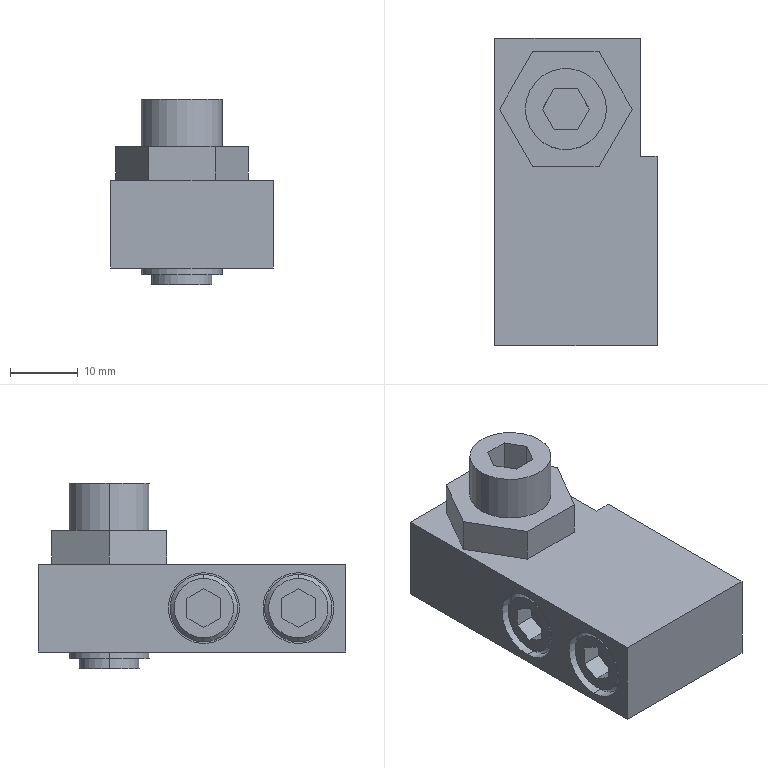Component | SolidWorks | SMC-MXS20-100AS-M9N-1_0SMC-MXS20-100AS-M9N-4-1 | 1 solid | 61 faces | box 24 x 45.5 x 27.5 mm | volume 15366 mm3 | plane 43 | cylinder 14 | cone 4 | commonest cylinder face diameters 10 x4 10.5 x4 12 x4 8.9 x2
build123d program:
from build123d import *

# Parameters (mm, degrees)
BOSS_EXTRUDE1_DEPTH      = 6.5
BOSS_EXTRUDE1_DEPTH_BACK = 6.5
SKETCH2_W                = 13
SKETCH2_H                = 6
CUT_EXTRUDE1_DEPTH       = 6
SKETCH5_R                = 6
BOSS_EXTRUDE2_DEPTH      = 5
SKETCH6_R                = 5.25
CUT_EXTRUDE2_DEPTH       = 6.5
SKETCH7_R                = 5.25
CUT_EXTRUDE3_DEPTH       = 6.5
CUT_EXTRUDE4_DEPTH       = 3
CUT_EXTRUDE5_DEPTH       = 3


with BuildPart() as part:
    # Sketch1 → Boss-Extrude1 (new, two sides: drawn at the far end of the back side and taken through both)
    with BuildSketch(Plane.XY.offset(-BOSS_EXTRUDE1_DEPTH_BACK)):
        Polygon((-24, 0), (0, 0), (0, 28), (-2.5, 28), (-2.5, 45.5), (-24, 45.5), align=None)
    extrude(amount=BOSS_EXTRUDE1_DEPTH + BOSS_EXTRUDE1_DEPTH_BACK)

    # Sketch2 → Cut-Revolve1 (revolve, cut)
    with BuildSketch(Plane(origin=(-13.5, 0, 0), x_dir=(0, 0, -1), z_dir=(1, 0, 0)), mode=Mode.PRIVATE) as cut_revolve1_sk:
        with Locations((0, 38)):
            Rectangle(SKETCH2_W, SKETCH2_H)
    revolve(cut_revolve1_sk.sketch.rotate(Axis((-13.5, 35, -6.5), (0, 0, 1)), 270), axis=Axis((-13.5, 35, -6.5), (0, 0, 1)), mode=Mode.SUBTRACT)

    # Sketch3 → Revolve1 (revolve)
    with BuildSketch(Plane(origin=(-13.5, 0, 0), x_dir=(0, 0, -1), z_dir=(1, 0, 0)), mode=Mode.PRIVATE) as revolve1_sk:
        Polygon((-18.5, 35), (-18.5, 41), (7.5, 41), (7.5, 39.45), (9, 39.45), (9, 35), align=None)
    revolve(revolve1_sk.sketch.rotate(Axis((-13.5, 35, -9), (0, 0, 1)), 270), axis=Axis((-13.5, 35, -9), (0, 0, 1)))

    # Sketch4 → Cut-Extrude1 (cut)
    with BuildSketch(Plane.XY.offset(18.5)):
        Polygon((-16.964, 35), (-15.232, 32), (-11.768, 32), (-10.036, 35), (-11.768, 38), (-15.232, 38), align=None)
    extrude(amount=-CUT_EXTRUDE1_DEPTH, mode=Mode.SUBTRACT)

    # Sketch5 → Boss-Extrude2 (add)
    with BuildSketch(Plane.XY.offset(6.5)):
        Polygon((-23.315, 35), (-18.407, 26.5), (-8.593, 26.5), (-3.685, 35), (-8.593, 43.5), (-18.407, 43.5), align=None)
        with Locations((-13.5, 35)):
            Circle(SKETCH5_R, mode=Mode.SUBTRACT)
    extrude(amount=BOSS_EXTRUDE2_DEPTH)

    # Sketch6 → Cut-Extrude2 (cut)
    with BuildSketch(Plane(origin=(-24, 0, 0), x_dir=(0, 0, -1), z_dir=(1, 0, 0))):
        with Locations((0, 7)):
            Circle(SKETCH6_R)
    extrude(amount=CUT_EXTRUDE2_DEPTH, mode=Mode.SUBTRACT)

    # Sketch7 → Cut-Extrude3 (cut)
    with BuildSketch(Plane(origin=(-24, 0, 0), x_dir=(0, 0, -1), z_dir=(1, 0, 0))):
        with Locations((0, 21)):
            Circle(SKETCH7_R)
    extrude(amount=CUT_EXTRUDE3_DEPTH, mode=Mode.SUBTRACT)

    # Sketch8 → Revolve2 (revolve)
    with BuildSketch(Plane.XY, mode=Mode.PRIVATE) as revolve2_sk:
        Polygon((-17.5, 7), (-17.5, 2), (-22.9, 2), (-23.5, 2.6), (-23.5, 7), align=None)
    revolve(revolve2_sk.sketch.rotate(Axis((-23.5, 7, 0), (1, 0, 0)), 90), axis=Axis((-23.5, 7, 0), (1, 0, 0)))

    # Sketch9 → Revolve3 (revolve)
    with BuildSketch(Plane.XY, mode=Mode.PRIVATE) as revolve3_sk:
        Polygon((-17.5, 21), (-17.5, 16), (-22.9, 16), (-23.5, 16.6), (-23.5, 21), align=None)
    revolve(revolve3_sk.sketch.rotate(Axis((-23.5, 21, 0), (1, 0, 0)), 90), axis=Axis((-23.5, 21, 0), (1, 0, 0)))

    # Sketch10 → Cut-Extrude4 (cut)
    with BuildSketch(Plane(origin=(-23.5, 0, 0), x_dir=(0, 0, -1), z_dir=(1, 0, 0))):
        Polygon((-2.887, 7), (-1.443, 4.5), (1.443, 4.5), (2.887, 7), (1.443, 9.5), (-1.443, 9.5), align=None)
    extrude(amount=CUT_EXTRUDE4_DEPTH, mode=Mode.SUBTRACT)

    # Sketch11 → Cut-Extrude5 (cut)
    with BuildSketch(Plane(origin=(-23.5, 0, 0), x_dir=(0, 0, -1), z_dir=(1, 0, 0))):
        Polygon((-2.887, 21), (-1.443, 18.5), (1.443, 18.5), (2.887, 21), (1.443, 23.5), (-1.443, 23.5), align=None)
    extrude(amount=CUT_EXTRUDE5_DEPTH, mode=Mode.SUBTRACT)


solid = part.part

# Placed as in the assembly
solid = solid.moved(Location((-271.509, 51.721, 134.089), (0, 0, 0)))